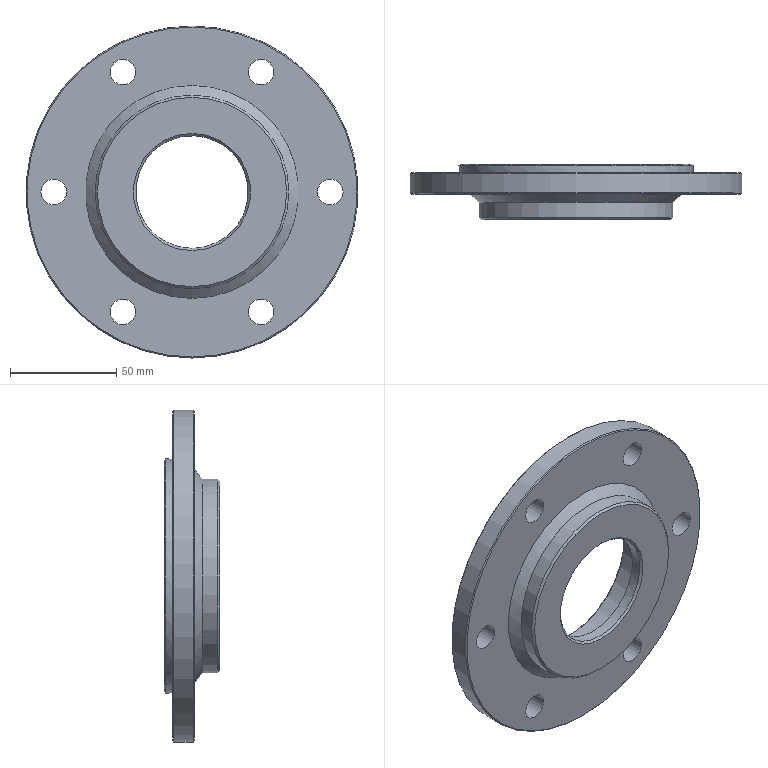Component | NX | SIDE_END_COVER_2 | 1 solid | 26 faces | volume 192724 mm3 | cylinder 12 | cone 8 | plane 6 | commonest cylinder face diameters 12 x6 53 x1 156 x1 91 x1 110 x1 100 x1 72 x1